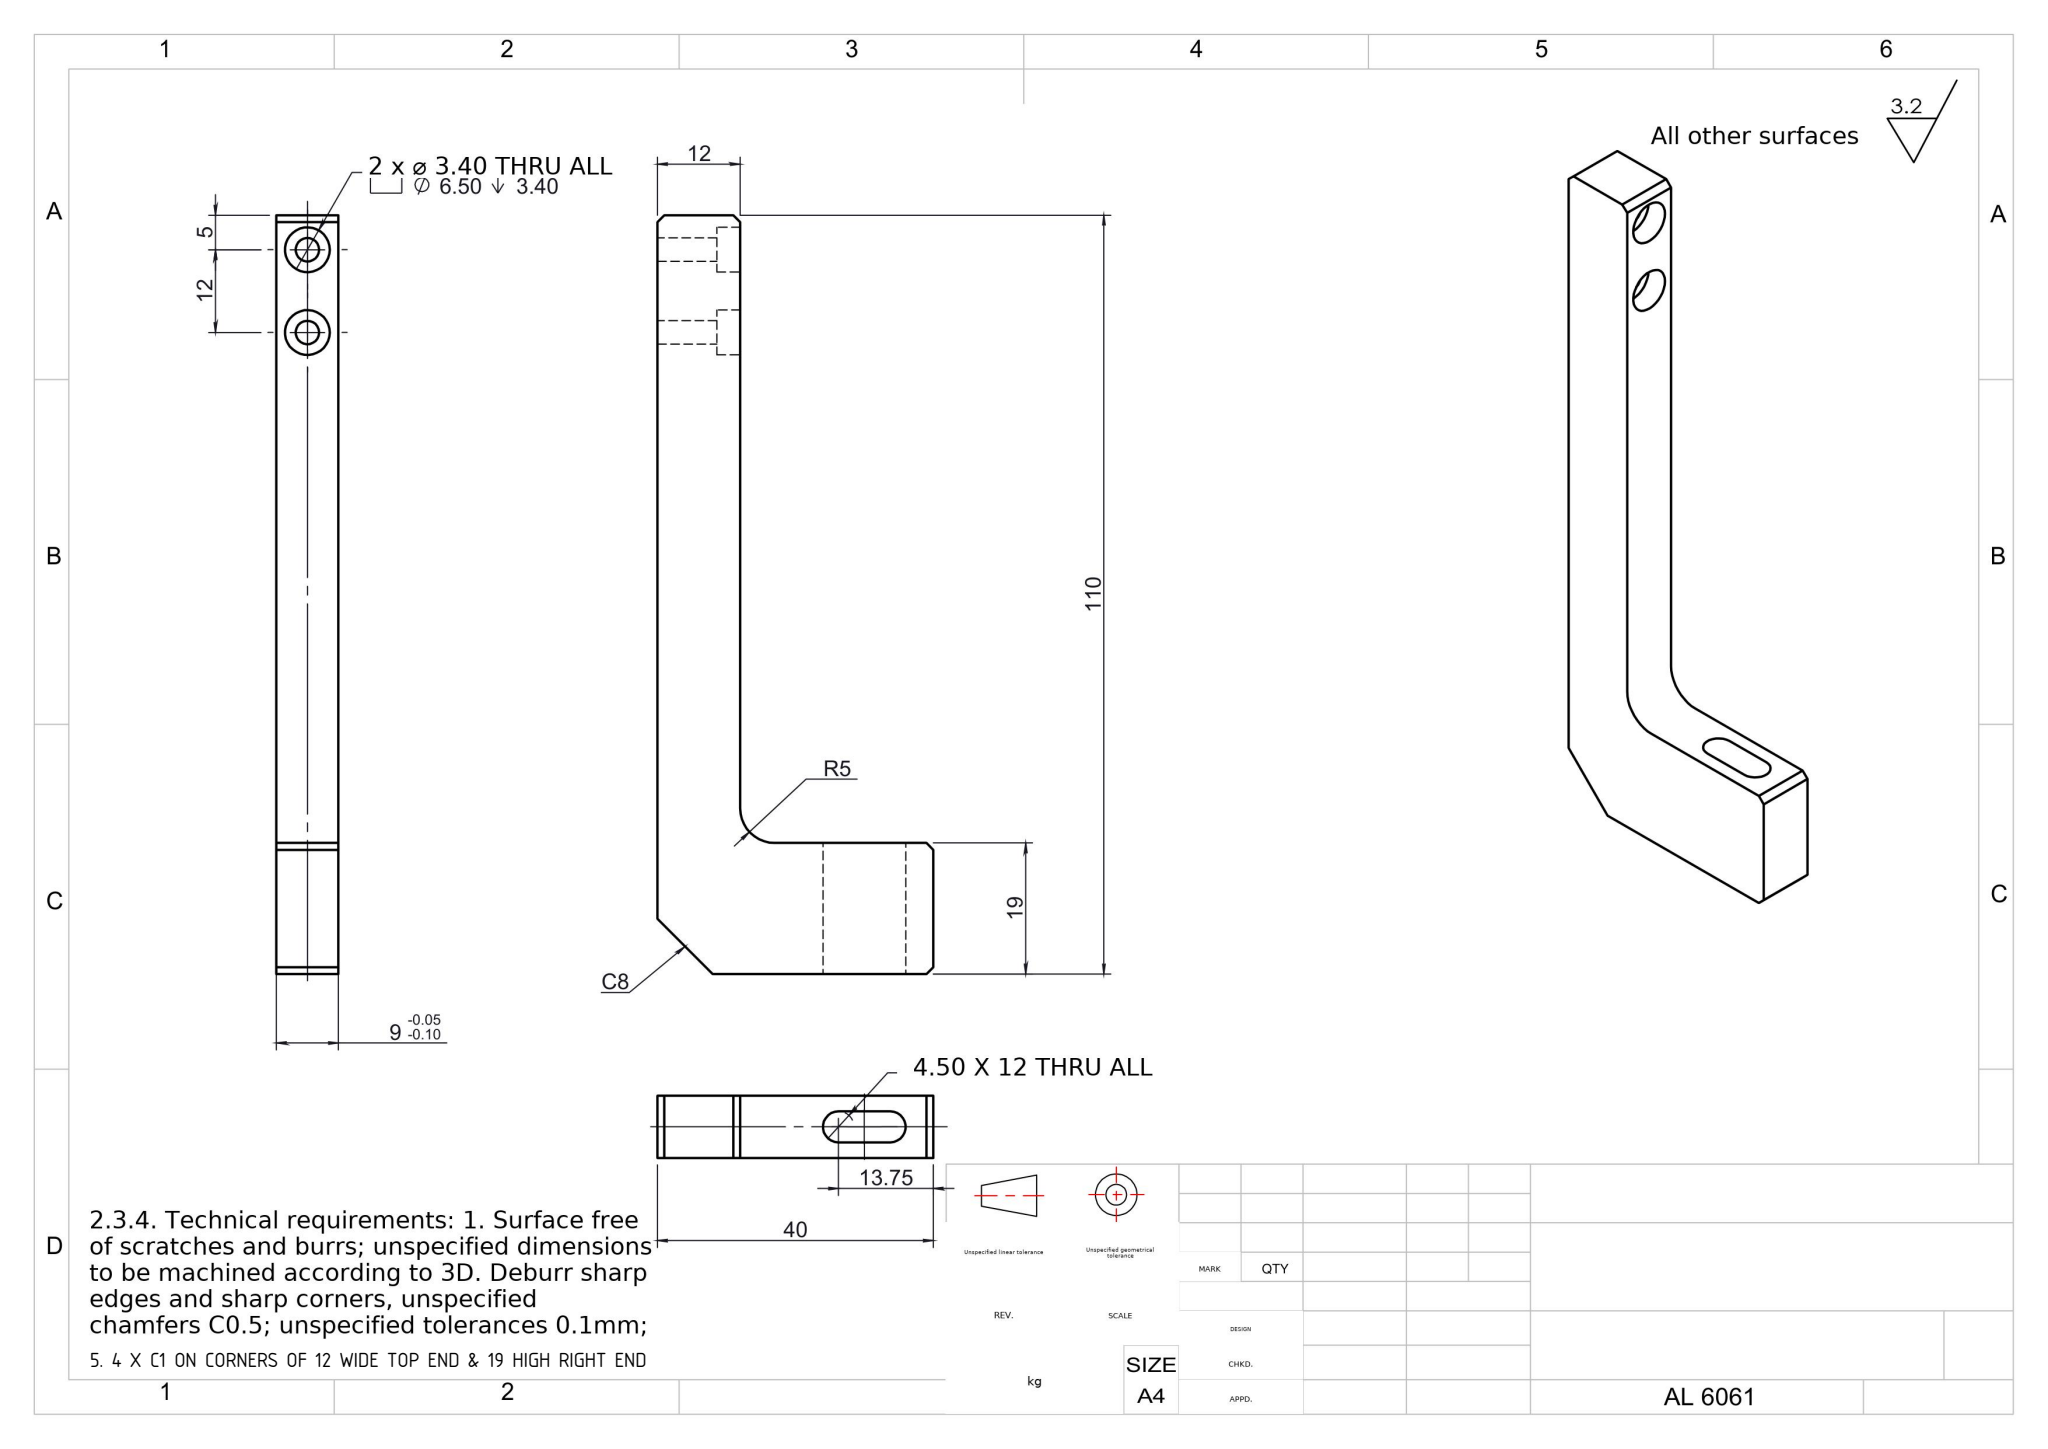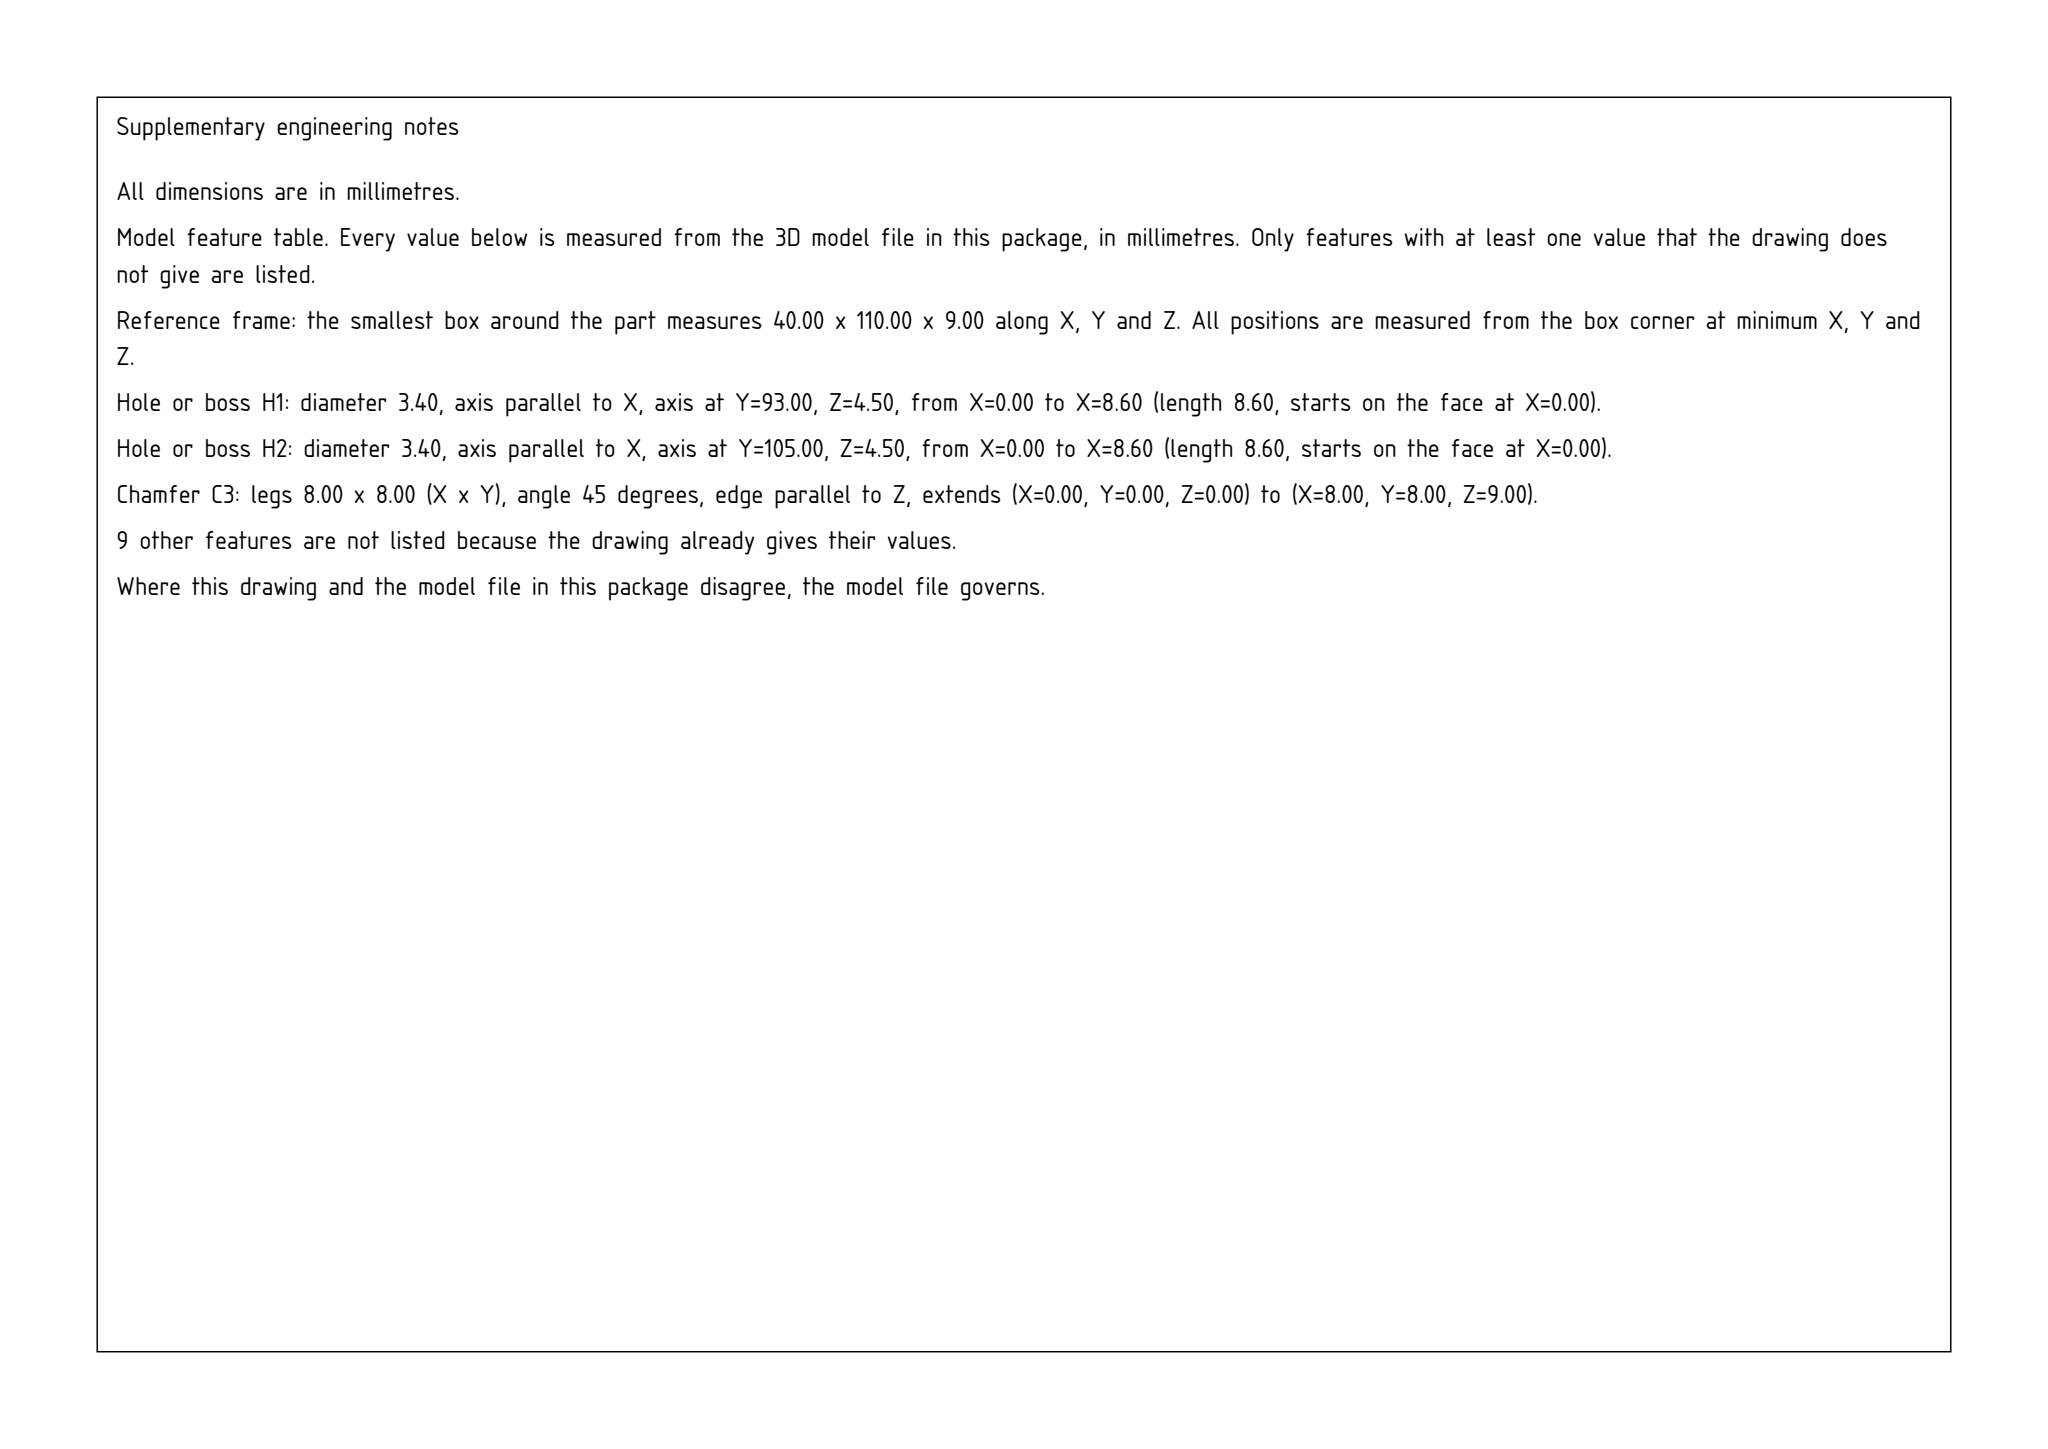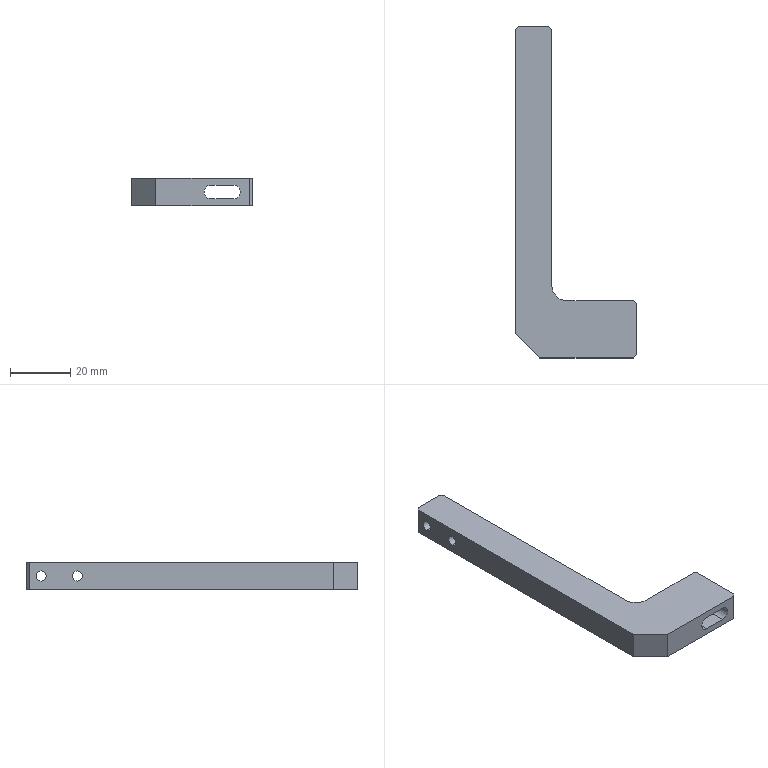Part | SolidWorks | mm | material AL 6061 | 1 solid | 28 faces | box 40 x 110 x 9 mm | volume 15085 mm3 | plane 17 | cylinder 11 | commonest cylinder face diameters 6.5 x4 3.4 x4 4.5 x2 10 x1
Drawing notes:
4 X C1 ON CORNERS OF 12 WIDE TOP END & 19 HIGH RIGHT END | from the solid: Four 45 deg inclined planes size 1x1x9 at [0,109,0], [11,109,0], [39,0,0], [39,18,0]; part bbox 40 x 110 x 9
STEP:
#1=CARTESIAN_POINT('',(-11.4,50.,3.25));
#2=VERTEX_POINT('',#1);
#3=CARTESIAN_POINT('',(-11.4,50.,-3.25));
#4=VERTEX_POINT('',#3);
#5=CARTESIAN_POINT('',(-11.4,50.,0.));
#6=DIRECTION('',(1.,0.,0.));
#7=DIRECTION('',(0.,0.,-1.));
#8=AXIS2_PLACEMENT_3D('',#5,#6,#7);
#9=CIRCLE('',#8,3.25);
#10=EDGE_CURVE('',#2,#4,#9,.T.);
#11=ORIENTED_EDGE('',*,*,#10,.F.);
#12=CARTESIAN_POINT('',(-8.,50.,3.25));
#13=VERTEX_POINT('',#12);
#14=CARTESIAN_POINT('',(-8.,50.,3.25));
#15=DIRECTION('',(1.,0.,0.));
#16=VECTOR('',#15,1000.);
#17=LINE('',#14,#16);
#18=EDGE_CURVE('',#2,#13,#17,.T.);
#19=ORIENTED_EDGE('',*,*,#18,.T.);
#20=CARTESIAN_POINT('',(-8.,50.,-3.25));
#21=VERTEX_POINT('',#20);
#22=CARTESIAN_POINT('',(-8.,50.,0.));
#23=DIRECTION('',(1.,0.,0.));
#24=DIRECTION('',(0.,0.,-1.));
#25=AXIS2_PLACEMENT_3D('',#22,#23,#24);
#26=CIRCLE('',#25,3.25);
#27=EDGE_CURVE('',#13,#21,#26,.T.);
#28=ORIENTED_EDGE('',*,*,#27,.T.);
#29=CARTESIAN_POINT('',(-8.,50.,-3.25));
#30=DIRECTION('',(1.,0.,0.));
#31=VECTOR('',#30,1000.);
#32=LINE('',#29,#31);
#33=EDGE_CURVE('',#4,#21,#32,.T.);
#34=ORIENTED_EDGE('',*,*,#33,.F.);
#35=EDGE_LOOP('',(#11,#19,#28,#34));
#36=FACE_OUTER_BOUND('',#35,.T.);
#37=CARTESIAN_POINT('',(-8.,50.,0.));
#38=DIRECTION('',(1.,0.,0.));
#39=DIRECTION('',(0.,0.,-1.));
#40=AXIS2_PLACEMENT_3D('',#37,#38,#39);
#41=CYLINDRICAL_SURFACE('',#40,3.25);
#42=ADVANCED_FACE('',(#36),#41,.F.);
#43=CARTESIAN_POINT('',(-20.,50.,1.7));
#44=VERTEX_POINT('',#43);
#45=CARTESIAN_POINT('',(-20.,50.,-1.7));
#46=VERTEX_POINT('',#45);
#47=CARTESIAN_POINT('',(-20.,50.,0.));
#48=DIRECTION('',(1.,0.,0.));
#49=DIRECTION('',(0.,0.,-1.));
#50=AXIS2_PLACEMENT_3D('',#47,#48,#49);
#51=CIRCLE('',#50,1.7);
#52=EDGE_CURVE('',#44,#46,#51,.T.);
#53=ORIENTED_EDGE('',*,*,#52,.F.);
#54=CARTESIAN_POINT('',(-11.4,50.,1.7));
#55=VERTEX_POINT('',#54);
#56=CARTESIAN_POINT('',(-8.,50.,1.7));
#57=DIRECTION('',(1.,0.,0.));
#58=VECTOR('',#57,1000.);
#59=LINE('',#56,#58);
#60=EDGE_CURVE('',#44,#55,#59,.T.);
#61=ORIENTED_EDGE('',*,*,#60,.T.);
#62=CARTESIAN_POINT('',(-11.4,50.,-1.7));
#63=VERTEX_POINT('',#62);
#64=CARTESIAN_POINT('',(-11.4,50.,0.));
#65=DIRECTION('',(1.,0.,0.));
#66=DIRECTION('',(0.,0.,-1.));
#67=AXIS2_PLACEMENT_3D('',#64,#65,#66);
#68=CIRCLE('',#67,1.7);
#69=EDGE_CURVE('',#55,#63,#68,.T.);
#70=ORIENTED_EDGE('',*,*,#69,.T.);
#71=CARTESIAN_POINT('',(-8.,50.,-1.7));
#72=DIRECTION('',(1.,0.,0.));
#73=VECTOR('',#72,1000.);
#74=LINE('',#71,#73);
#75=EDGE_CURVE('',#46,#63,#74,.T.);
#76=ORIENTED_EDGE('',*,*,#75,.F.);
#77=EDGE_LOOP('',(#53,#61,#70,#76));
#78=FACE_OUTER_BOUND('',#77,.T.);
#79=CARTESIAN_POINT('',(-8.,50.,0.));
#80=DIRECTION('',(1.,0.,0.));
#81=DIRECTION('',(0.,0.,-1.));
#82=AXIS2_PLACEMENT_3D('',#79,#80,#81);
#83=CYLINDRICAL_SURFACE('',#82,1.7);
#84=ADVANCED_FACE('',(#78),#83,.F.);
#85=CARTESIAN_POINT('',(-11.4,38.,3.25));
#86=VERTEX_POINT('',#85);
#87=CARTESIAN_POINT('',(-11.4,38.,-3.25));
#88=VERTEX_POINT('',#87);
#89=CARTESIAN_POINT('',(-11.4,38.,0.));
#90=DIRECTION('',(1.,0.,0.));
#91=DIRECTION('',(0.,0.,-1.));
#92=AXIS2_PLACEMENT_3D('',#89,#90,#91);
#93=CIRCLE('',#92,3.25);
#94=EDGE_CURVE('',#86,#88,#93,.T.);
#95=ORIENTED_EDGE('',*,*,#94,.F.);
#96=CARTESIAN_POINT('',(-8.,38.,3.25));
#97=VERTEX_POINT('',#96);
#98=CARTESIAN_POINT('',(-8.,38.,3.25));
#99=DIRECTION('',(1.,0.,0.));
#100=VECTOR('',#99,1000.);
#101=LINE('',#98,#100);
#102=EDGE_CURVE('',#86,#97,#101,.T.);
#103=ORIENTED_EDGE('',*,*,#102,.T.);
#104=CARTESIAN_POINT('',(-8.,38.,-3.25));
#105=VERTEX_POINT('',#104);
#106=CARTESIAN_POINT('',(-8.,38.,0.));
#107=DIRECTION('',(1.,0.,0.));
#108=DIRECTION('',(0.,0.,-1.));
#109=AXIS2_PLACEMENT_3D('',#106,#107,#108);
#110=CIRCLE('',#109,3.25);
#111=EDGE_CURVE('',#97,#105,#110,.T.);
#112=ORIENTED_EDGE('',*,*,#111,.T.);
#113=CARTESIAN_POINT('',(-8.,38.,-3.25));
#114=DIRECTION('',(1.,0.,0.));
#115=VECTOR('',#114,1000.);
#116=LINE('',#113,#115);
#117=EDGE_CURVE('',#88,#105,#116,.T.);
#118=ORIENTED_EDGE('',*,*,#117,.F.);
#119=EDGE_LOOP('',(#95,#103,#112,#118));
#120=FACE_OUTER_BOUND('',#119,.T.);
#121=CARTESIAN_POINT('',(-8.,38.,0.));
#122=DIRECTION('',(1.,0.,0.));
#123=DIRECTION('',(0.,0.,-1.));
#124=AXIS2_PLACEMENT_3D('',#121,#122,#123);
#125=CYLINDRICAL_SURFACE('',#124,3.25);
#126=ADVANCED_FACE('',(#120),#125,.F.);
#127=CARTESIAN_POINT('',(-20.,38.,1.7));
#128=VERTEX_POINT('',#127);
#129=CARTESIAN_POINT('',(-20.,38.,-1.7));
#130=VERTEX_POINT('',#129);
#131=CARTESIAN_POINT('',(-20.,38.,0.));
#132=DIRECTION('',(1.,0.,0.));
#133=DIRECTION('',(0.,0.,-1.));
#134=AXIS2_PLACEMENT_3D('',#131,#132,#133);
#135=CIRCLE('',#134,1.7);
#136=EDGE_CURVE('',#128,#130,#135,.T.);
#137=ORIENTED_EDGE('',*,*,#136,.F.);
#138=CARTESIAN_POINT('',(-11.4,38.,1.7));
#139=VERTEX_POINT('',#138);
#140=CARTESIAN_POINT('',(-8.,38.,1.7));
#141=DIRECTION('',(1.,0.,0.));
#142=VECTOR('',#141,1000.);
#143=LINE('',#140,#142);
#144=EDGE_CURVE('',#128,#139,#143,.T.);
#145=ORIENTED_EDGE('',*,*,#144,.T.);
#146=CARTESIAN_POINT('',(-11.4,38.,-1.7));
#147=VERTEX_POINT('',#146);
#148=CARTESIAN_POINT('',(-11.4,38.,0.));
#149=DIRECTION('',(1.,0.,0.));
#150=DIRECTION('',(0.,0.,-1.));
#151=AXIS2_PLACEMENT_3D('',#148,#149,#150);
#152=CIRCLE('',#151,1.7);
#153=EDGE_CURVE('',#139,#147,#152,.T.);
#154=ORIENTED_EDGE('',*,*,#153,.T.);
#155=CARTESIAN_POINT('',(-8.,38.,-1.7));
#156=DIRECTION('',(1.,0.,0.));
#157=VECTOR('',#156,1000.);
#158=LINE('',#155,#157);
#159=EDGE_CURVE('',#130,#147,#158,.T.);
#160=ORIENTED_EDGE('',*,*,#159,.F.);
#161=EDGE_LOOP('',(#137,#145,#154,#160));
#162=FACE_OUTER_BOUND('',#161,.T.);
#163=CARTESIAN_POINT('',(-8.,38.,0.));
#164=DIRECTION('',(1.,0.,0.));
#165=DIRECTION('',(0.,0.,-1.));
#166=AXIS2_PLACEMENT_3D('',#163,#164,#165);
#167=CYLINDRICAL_SURFACE('',#166,1.7);
#168=ADVANCED_FACE('',(#162),#167,.F.);
#169=CARTESIAN_POINT('',(-20.,50.,0.));
#170=DIRECTION('',(1.,0.,0.));
#171=DIRECTION('',(0.,0.,-1.));
#172=AXIS2_PLACEMENT_3D('',#169,#170,#171);
#173=CIRCLE('',#172,1.7);
#174=EDGE_CURVE('',#46,#44,#173,.T.);
#175=ORIENTED_EDGE('',*,*,#174,.T.);
#176=ORIENTED_EDGE('',*,*,#52,.T.);
#177=EDGE_LOOP('',(#175,#176));
#178=FACE_BOUND('',#177,.T.);
#179=CARTESIAN_POINT('',(-20.,38.,0.));
#180=DIRECTION('',(1.,0.,0.));
#181=DIRECTION('',(0.,0.,-1.));
#182=AXIS2_PLACEMENT_3D('',#179,#180,#181);
#183=CIRCLE('',#182,1.7);
#184=EDGE_CURVE('',#130,#128,#183,.T.);
#185=ORIENTED_EDGE('',*,*,#184,.T.);
#186=ORIENTED_EDGE('',*,*,#136,.T.);
#187=EDGE_LOOP('',(#185,#186));
#188=FACE_BOUND('',#187,.T.);
#189=CARTESIAN_POINT('',(-20.,54.,4.5));
#190=VERTEX_POINT('',#189);
#191=CARTESIAN_POINT('',(-20.,-47.,4.5));
#192=VERTEX_POINT('',#191);
#193=CARTESIAN_POINT('',(-20.,-55.,4.5));
#194=DIRECTION('',(0.,-1.,0.));
#195=VECTOR('',#194,1000.);
#196=LINE('',#193,#195);
#197=EDGE_CURVE('',#190,#192,#196,.T.);
#198=ORIENTED_EDGE('',*,*,#197,.F.);
#199=CARTESIAN_POINT('',(-20.,54.,-4.5));
#200=VERTEX_POINT('',#199);
#201=CARTESIAN_POINT('',(-20.,54.,4.5));
#202=DIRECTION('',(0.,0.,-1.));
#203=VECTOR('',#202,1000.);
#204=LINE('',#201,#203);
#205=EDGE_CURVE('',#190,#200,#204,.T.);
#206=ORIENTED_EDGE('',*,*,#205,.T.);
#207=CARTESIAN_POINT('',(-20.,-47.,-4.5));
#208=VERTEX_POINT('',#207);
#209=CARTESIAN_POINT('',(-20.,-55.,-4.5));
#210=DIRECTION('',(0.,-1.,0.));
#211=VECTOR('',#210,1000.);
#212=LINE('',#209,#211);
#213=EDGE_CURVE('',#200,#208,#212,.T.);
#214=ORIENTED_EDGE('',*,*,#213,.T.);
#215=CARTESIAN_POINT('',(-20.,-47.,4.5));
#216=DIRECTION('',(0.,0.,1.));
#217=VECTOR('',#216,1000.);
#218=LINE('',#215,#217);
#219=EDGE_CURVE('',#208,#192,#218,.T.);
#220=ORIENTED_EDGE('',*,*,#219,.T.);
#221=EDGE_LOOP('',(#198,#206,#214,#220));
#222=FACE_OUTER_BOUND('',#221,.T.);
#223=CARTESIAN_POINT('',(-20.,-55.,4.5));
#224=DIRECTION('',(1.,0.,0.));
#225=DIRECTION('',(0.,0.,-1.));
#226=AXIS2_PLACEMENT_3D('',#223,#224,#225);
#227=PLANE('',#226);
#228=ADVANCED_FACE('',(#178,#188,#222),#227,.F.);
#229=CARTESIAN_POINT('',(6.25,-55.,-2.25));
#230=VERTEX_POINT('',#229);
#231=CARTESIAN_POINT('',(6.25,-55.,2.25));
#232=VERTEX_POINT('',#231);
#233=CARTESIAN_POINT('',(6.25,-55.,-0.));
#234=DIRECTION('',(0.,1.,0.));
#235=DIRECTION('',(0.,0.,1.));
#236=AXIS2_PLACEMENT_3D('',#233,#234,#235);
#237=CIRCLE('',#236,2.25);
#238=EDGE_CURVE('',#230,#232,#237,.T.);
#239=ORIENTED_EDGE('',*,*,#238,.T.);
#240=CARTESIAN_POINT('',(13.75,-55.,2.25));
#241=VERTEX_POINT('',#240);
#242=CARTESIAN_POINT('',(6.25,-55.,2.25));
#243=DIRECTION('',(1.,0.,-0.));
#244=VECTOR('',#243,1000.);
#245=LINE('',#242,#244);
#246=EDGE_CURVE('',#232,#241,#245,.T.);
#247=ORIENTED_EDGE('',*,*,#246,.T.);
#248=CARTESIAN_POINT('',(13.75,-55.,-2.25));
#249=VERTEX_POINT('',#248);
#250=CARTESIAN_POINT('',(13.75,-55.,-0.));
#251=DIRECTION('',(0.,1.,0.));
#252=DIRECTION('',(0.,0.,1.));
#253=AXIS2_PLACEMENT_3D('',#250,#251,#252);
#254=CIRCLE('',#253,2.25);
#255=EDGE_CURVE('',#241,#249,#254,.T.);
#256=ORIENTED_EDGE('',*,*,#255,.T.);
#257=CARTESIAN_POINT('',(6.25,-55.,-2.25));
#258=DIRECTION('',(1.,0.,-0.));
#259=VECTOR('',#258,1000.);
#260=LINE('',#257,#259);
#261=EDGE_CURVE('',#230,#249,#260,.T.);
#262=ORIENTED_EDGE('',*,*,#261,.F.);
#263=EDGE_LOOP('',(#239,#247,#256,#262));
#264=FACE_BOUND('',#263,.T.);
#265=CARTESIAN_POINT('',(-12.,-55.,-4.5));
#266=VERTEX_POINT('',#265);
#267=CARTESIAN_POINT('',(19.,-55.,-4.5));
#268=VERTEX_POINT('',#267);
#269=CARTESIAN_POINT('',(20.,-55.,-4.5));
#270=DIRECTION('',(1.,0.,0.));
#271=VECTOR('',#270,1000.);
#272=LINE('',#269,#271);
#273=EDGE_CURVE('',#266,#268,#272,.T.);
#274=ORIENTED_EDGE('',*,*,#273,.T.);
#275=CARTESIAN_POINT('',(19.,-55.,4.5));
#276=VERTEX_POINT('',#275);
#277=CARTESIAN_POINT('',(19.,-55.,4.5));
#278=DIRECTION('',(0.,0.,1.));
#279=VECTOR('',#278,1000.);
#280=LINE('',#277,#279);
#281=EDGE_CURVE('',#268,#276,#280,.T.);
#282=ORIENTED_EDGE('',*,*,#281,.T.);
#283=CARTESIAN_POINT('',(-12.,-55.,4.5));
#284=VERTEX_POINT('',#283);
#285=CARTESIAN_POINT('',(20.,-55.,4.5));
#286=DIRECTION('',(1.,0.,0.));
#287=VECTOR('',#286,1000.);
#288=LINE('',#285,#287);
#289=EDGE_CURVE('',#284,#276,#288,.T.);
#290=ORIENTED_EDGE('',*,*,#289,.F.);
#291=CARTESIAN_POINT('',(-12.,-55.,4.5));
#292=DIRECTION('',(0.,0.,-1.));
#293=VECTOR('',#292,1000.);
#294=LINE('',#291,#293);
#295=EDGE_CURVE('',#284,#266,#294,.T.);
#296=ORIENTED_EDGE('',*,*,#295,.T.);
#297=EDGE_LOOP('',(#274,#282,#290,#296));
#298=FACE_OUTER_BOUND('',#297,.T.);
#299=CARTESIAN_POINT('',(20.,-55.,4.5));
#300=DIRECTION('',(0.,1.,0.));
#301=DIRECTION('',(0.,0.,1.));
#302=AXIS2_PLACEMENT_3D('',#299,#300,#301);
#303=PLANE('',#302);
#304=ADVANCED_FACE('',(#264,#298),#303,.F.);
#305=CARTESIAN_POINT('',(20.,-54.,4.5));
#306=VERTEX_POINT('',#305);
#307=CARTESIAN_POINT('',(20.,-37.,4.5));
#308=VERTEX_POINT('',#307);
#309=CARTESIAN_POINT('',(20.,-55.,4.5));
#310=DIRECTION('',(0.,1.,0.));
#311=VECTOR('',#310,1000.);
#312=LINE('',#309,#311);
#313=EDGE_CURVE('',#306,#308,#312,.T.);
#314=ORIENTED_EDGE('',*,*,#313,.F.);
#315=CARTESIAN_POINT('',(20.,-54.,-4.5));
#316=VERTEX_POINT('',#315);
#317=CARTESIAN_POINT('',(20.,-54.,4.5));
#318=DIRECTION('',(0.,0.,-1.));
#319=VECTOR('',#318,1000.);
#320=LINE('',#317,#319);
#321=EDGE_CURVE('',#306,#316,#320,.T.);
#322=ORIENTED_EDGE('',*,*,#321,.T.);
#323=CARTESIAN_POINT('',(20.,-37.,-4.5));
#324=VERTEX_POINT('',#323);
#325=CARTESIAN_POINT('',(20.,-55.,-4.5));
#326=DIRECTION('',(0.,1.,0.));
#327=VECTOR('',#326,1000.);
#328=LINE('',#325,#327);
#329=EDGE_CURVE('',#316,#324,#328,.T.);
#330=ORIENTED_EDGE('',*,*,#329,.T.);
#331=CARTESIAN_POINT('',(20.,-37.,4.5));
#332=DIRECTION('',(0.,0.,1.));
#333=VECTOR('',#332,1000.);
#334=LINE('',#331,#333);
#335=EDGE_CURVE('',#324,#308,#334,.T.);
#336=ORIENTED_EDGE('',*,*,#335,.T.);
#337=EDGE_LOOP('',(#314,#322,#330,#336));
#338=FACE_OUTER_BOUND('',#337,.T.);
#339=CARTESIAN_POINT('',(20.,-55.,4.5));
#340=DIRECTION('',(-1.,0.,0.));
#341=DIRECTION('',(0.,0.,1.));
#342=AXIS2_PLACEMENT_3D('',#339,#340,#341);
#343=PLANE('',#342);
#344=ADVANCED_FACE('',(#338),#343,.F.);
#345=CARTESIAN_POINT('',(-9.,55.,-4.5));
#346=VERTEX_POINT('',#345);
#347=CARTESIAN_POINT('',(-19.,55.,-4.5));
#348=VERTEX_POINT('',#347);
#349=CARTESIAN_POINT('',(20.,55.,-4.5));
#350=DIRECTION('',(-1.,0.,0.));
#351=VECTOR('',#350,1000.);
#352=LINE('',#349,#351);
#353=EDGE_CURVE('',#346,#348,#352,.T.);
#354=ORIENTED_EDGE('',*,*,#353,.T.);
#355=CARTESIAN_POINT('',(-19.,55.,4.5));
#356=VERTEX_POINT('',#355);
#357=CARTESIAN_POINT('',(-19.,55.,4.5));
#358=DIRECTION('',(0.,0.,1.));
#359=VECTOR('',#358,1000.);
#360=LINE('',#357,#359);
#361=EDGE_CURVE('',#348,#356,#360,.T.);
#362=ORIENTED_EDGE('',*,*,#361,.T.);
#363=CARTESIAN_POINT('',(-9.,55.,4.5));
#364=VERTEX_POINT('',#363);
#365=CARTESIAN_POINT('',(20.,55.,4.5));
#366=DIRECTION('',(-1.,0.,0.));
#367=VECTOR('',#366,1000.);
#368=LINE('',#365,#367);
#369=EDGE_CURVE('',#364,#356,#368,.T.);
#370=ORIENTED_EDGE('',*,*,#369,.F.);
#371=CARTESIAN_POINT('',(-9.,55.,4.5));
#372=DIRECTION('',(0.,0.,-1.));
#373=VECTOR('',#372,1000.);
#374=LINE('',#371,#373);
#375=EDGE_CURVE('',#364,#346,#374,.T.);
#376=ORIENTED_EDGE('',*,*,#375,.T.);
#377=EDGE_LOOP('',(#354,#362,#370,#376));
#378=FACE_OUTER_BOUND('',#377,.T.);
#379=CARTESIAN_POINT('',(20.,55.,4.5));
#380=DIRECTION('',(0.,-1.,0.));
#381=DIRECTION('',(0.,0.,-1.));
#382=AXIS2_PLACEMENT_3D('',#379,#380,#381);
#383=PLANE('',#382);
#384=ADVANCED_FACE('',(#378),#383,.F.);
#385=ORIENTED_EDGE('',*,*,#289,.T.);
#386=CARTESIAN_POINT('',(37.,-37.,4.5));
#387=DIRECTION('',(0.7071,0.7071,0.));
#388=VECTOR('',#387,1000.);
#389=LINE('',#386,#388);
#390=EDGE_CURVE('',#276,#306,#389,.T.);
#391=ORIENTED_EDGE('',*,*,#390,.T.);
#392=ORIENTED_EDGE('',*,*,#313,.T.);
#393=CARTESIAN_POINT('',(19.,-36.,4.5));
#394=VERTEX_POINT('',#393);
#395=CARTESIAN_POINT('',(-8.5,-8.5,4.5));
#396=DIRECTION('',(-0.7071,0.7071,0.));
#397=VECTOR('',#396,1000.);
#398=LINE('',#395,#397);
#399=EDGE_CURVE('',#308,#394,#398,.T.);
#400=ORIENTED_EDGE('',*,*,#399,.T.);
#401=CARTESIAN_POINT('',(-3.,-36.,4.5));
#402=VERTEX_POINT('',#401);
#403=CARTESIAN_POINT('',(20.,-36.,4.5));
#404=DIRECTION('',(1.,0.,0.));
#405=VECTOR('',#404,1000.);
#406=LINE('',#403,#405);
#407=EDGE_CURVE('',#402,#394,#406,.T.);
#408=ORIENTED_EDGE('',*,*,#407,.F.);
#409=CARTESIAN_POINT('',(-8.,-31.,4.5));
#410=VERTEX_POINT('',#409);
#411=CARTESIAN_POINT('',(-3.,-31.,4.5));
#412=DIRECTION('',(0.,0.,-1.));
#413=DIRECTION('',(1.,0.,0.));
#414=AXIS2_PLACEMENT_3D('',#411,#412,#413);
#415=CIRCLE('',#414,5.);
#416=EDGE_CURVE('',#402,#410,#415,.T.);
#417=ORIENTED_EDGE('',*,*,#416,.T.);
#418=CARTESIAN_POINT('',(-8.,54.,4.5));
#419=VERTEX_POINT('',#418);
#420=CARTESIAN_POINT('',(-8.,55.,4.5));
#421=DIRECTION('',(0.,-1.,0.));
#422=VECTOR('',#421,1000.);
#423=LINE('',#420,#422);
#424=EDGE_CURVE('',#419,#410,#423,.T.);
#425=ORIENTED_EDGE('',*,*,#424,.F.);
#426=CARTESIAN_POINT('',(23.,23.,4.5));
#427=DIRECTION('',(-0.7071,0.7071,0.));
#428=VECTOR('',#427,1000.);
#429=LINE('',#426,#428);
#430=EDGE_CURVE('',#419,#364,#429,.T.);
#431=ORIENTED_EDGE('',*,*,#430,.T.);
#432=ORIENTED_EDGE('',*,*,#369,.T.);
#433=CARTESIAN_POINT('',(-37.,37.,4.5));
#434=DIRECTION('',(-0.7071,-0.7071,0.));
#435=VECTOR('',#434,1000.);
#436=LINE('',#433,#435);
#437=EDGE_CURVE('',#356,#190,#436,.T.);
#438=ORIENTED_EDGE('',*,*,#437,.T.);
#439=ORIENTED_EDGE('',*,*,#197,.T.);
#440=CARTESIAN_POINT('',(-33.5,-33.5,4.5));
#441=DIRECTION('',(0.7071,-0.7071,0.));
#442=VECTOR('',#441,1000.);
#443=LINE('',#440,#442);
#444=EDGE_CURVE('',#192,#284,#443,.T.);
#445=ORIENTED_EDGE('',*,*,#444,.T.);
#446=EDGE_LOOP('',(#385,#391,#392,#400,#408,#417,#425,#431,#432,#438,#439,#445));
#447=FACE_OUTER_BOUND('',#446,.T.);
#448=CARTESIAN_POINT('',(0.,0.,4.5));
#449=DIRECTION('',(0.,0.,1.));
#450=DIRECTION('',(1.,0.,0.));
#451=AXIS2_PLACEMENT_3D('',#448,#449,#450);
#452=PLANE('',#451);
#453=ADVANCED_FACE('',(#447),#452,.T.);
#454=ORIENTED_EDGE('',*,*,#329,.F.);
#455=CARTESIAN_POINT('',(20.,-54.,-4.5));
#456=DIRECTION('',(-0.7071,-0.7071,0.));
#457=VECTOR('',#456,1000.);
#458=LINE('',#455,#457);
#459=EDGE_CURVE('',#316,#268,#458,.T.);
#460=ORIENTED_EDGE('',*,*,#459,.T.);
#461=ORIENTED_EDGE('',*,*,#273,.F.);
#462=CARTESIAN_POINT('',(-12.,-55.,-4.5));
#463=DIRECTION('',(-0.7071,0.7071,0.));
#464=VECTOR('',#463,1000.);
#465=LINE('',#462,#464);
#466=EDGE_CURVE('',#266,#208,#465,.T.);
#467=ORIENTED_EDGE('',*,*,#466,.T.);
#468=ORIENTED_EDGE('',*,*,#213,.F.);
#469=CARTESIAN_POINT('',(-20.,54.,-4.5));
#470=DIRECTION('',(0.7071,0.7071,0.));
#471=VECTOR('',#470,1000.);
#472=LINE('',#469,#471);
#473=EDGE_CURVE('',#200,#348,#472,.T.);
#474=ORIENTED_EDGE('',*,*,#473,.T.);
#475=ORIENTED_EDGE('',*,*,#353,.F.);
#476=CARTESIAN_POINT('',(-8.,54.,-4.5));
#477=VERTEX_POINT('',#476);
#478=CARTESIAN_POINT('',(-8.,54.,-4.5));
#479=DIRECTION('',(0.7071,-0.7071,0.));
#480=VECTOR('',#479,1000.);
#481=LINE('',#478,#480);
#482=EDGE_CURVE('',#346,#477,#481,.T.);
#483=ORIENTED_EDGE('',*,*,#482,.T.);
#484=CARTESIAN_POINT('',(-8.,-31.,-4.5));
#485=VERTEX_POINT('',#484);
#486=CARTESIAN_POINT('',(-8.,55.,-4.5));
#487=DIRECTION('',(0.,-1.,0.));
#488=VECTOR('',#487,1000.);
#489=LINE('',#486,#488);
#490=EDGE_CURVE('',#477,#485,#489,.T.);
#491=ORIENTED_EDGE('',*,*,#490,.T.);
#492=CARTESIAN_POINT('',(-3.,-36.,-4.5));
#493=VERTEX_POINT('',#492);
#494=CARTESIAN_POINT('',(-3.,-31.,-4.5));
#495=DIRECTION('',(0.,0.,1.));
#496=DIRECTION('',(1.,0.,0.));
#497=AXIS2_PLACEMENT_3D('',#494,#495,#496);
#498=CIRCLE('',#497,5.);
#499=EDGE_CURVE('',#485,#493,#498,.T.);
#500=ORIENTED_EDGE('',*,*,#499,.T.);
#501=CARTESIAN_POINT('',(19.,-36.,-4.5));
#502=VERTEX_POINT('',#501);
#503=CARTESIAN_POINT('',(20.,-36.,-4.5));
#504=DIRECTION('',(1.,0.,0.));
#505=VECTOR('',#504,1000.);
#506=LINE('',#503,#505);
#507=EDGE_CURVE('',#493,#502,#506,.T.);
#508=ORIENTED_EDGE('',*,*,#507,.T.);
#509=CARTESIAN_POINT('',(20.,-37.,-4.5));
#510=DIRECTION('',(0.7071,-0.7071,0.));
#511=VECTOR('',#510,1000.);
#512=LINE('',#509,#511);
#513=EDGE_CURVE('',#502,#324,#512,.T.);
#514=ORIENTED_EDGE('',*,*,#513,.T.);
#515=EDGE_LOOP('',(#454,#460,#461,#467,#468,#474,#475,#483,#491,#500,#508,#514));
#516=FACE_OUTER_BOUND('',#515,.T.);
#517=CARTESIAN_POINT('',(0.,0.,-4.5));
#518=DIRECTION('',(0.,0.,1.));
#519=DIRECTION('',(1.,0.,0.));
#520=AXIS2_PLACEMENT_3D('',#517,#518,#519);
#521=PLANE('',#520);
#522=ADVANCED_FACE('',(#516),#521,.F.);
#523=CARTESIAN_POINT('',(6.25,-36.,-2.25));
#524=VERTEX_POINT('',#523);
#525=CARTESIAN_POINT('',(6.25,-36.,2.25));
#526=VERTEX_POINT('',#525);
#527=CARTESIAN_POINT('',(6.25,-36.,-0.));
#528=DIRECTION('',(0.,1.,0.));
#529=DIRECTION('',(0.,0.,1.));
#530=AXIS2_PLACEMENT_3D('',#527,#528,#529);
#531=CIRCLE('',#530,2.25);
#532=EDGE_CURVE('',#524,#526,#531,.T.);
#533=ORIENTED_EDGE('',*,*,#532,.F.);
#534=CARTESIAN_POINT('',(13.75,-36.,-2.25));
#535=VERTEX_POINT('',#534);
#536=CARTESIAN_POINT('',(6.25,-36.,-2.25));
#537=DIRECTION('',(1.,0.,-0.));
#538=VECTOR('',#537,1000.);
#539=LINE('',#536,#538);
#540=EDGE_CURVE('',#524,#535,#539,.T.);
#541=ORIENTED_EDGE('',*,*,#540,.T.);
#542=CARTESIAN_POINT('',(13.75,-36.,2.25));
#543=VERTEX_POINT('',#542);
#544=CARTESIAN_POINT('',(13.75,-36.,-0.));
#545=DIRECTION('',(0.,1.,0.));
#546=DIRECTION('',(0.,0.,1.));
#547=AXIS2_PLACEMENT_3D('',#544,#545,#546);
#548=CIRCLE('',#547,2.25);
#549=EDGE_CURVE('',#543,#535,#548,.T.);
#550=ORIENTED_EDGE('',*,*,#549,.F.);
#551=CARTESIAN_POINT('',(6.25,-36.,2.25));
#552=DIRECTION('',(1.,0.,-0.));
#553=VECTOR('',#552,1000.);
#554=LINE('',#551,#553);
#555=EDGE_CURVE('',#526,#543,#554,.T.);
#556=ORIENTED_EDGE('',*,*,#555,.F.);
#557=EDGE_LOOP('',(#533,#541,#550,#556));
#558=FACE_BOUND('',#557,.T.);
#559=ORIENTED_EDGE('',*,*,#407,.T.);
#560=CARTESIAN_POINT('',(19.,-36.,-4.5));
#561=DIRECTION('',(0.,0.,-1.));
#562=VECTOR('',#561,1000.);
#563=LINE('',#560,#562);
#564=EDGE_CURVE('',#394,#502,#563,.T.);
#565=ORIENTED_EDGE('',*,*,#564,.T.);
#566=ORIENTED_EDGE('',*,*,#507,.F.);
#567=CARTESIAN_POINT('',(-3.,-36.,4.5));
#568=DIRECTION('',(0.,0.,1.));
#569=VECTOR('',#568,1000.);
#570=LINE('',#567,#569);
#571=EDGE_CURVE('',#493,#402,#570,.T.);
#572=ORIENTED_EDGE('',*,*,#571,.T.);
#573=EDGE_LOOP('',(#559,#565,#566,#572));
#574=FACE_OUTER_BOUND('',#573,.T.);
#575=CARTESIAN_POINT('',(20.,-36.,-4.5));
#576=DIRECTION('',(0.,-1.,0.));
#577=DIRECTION('',(0.,0.,-1.));
#578=AXIS2_PLACEMENT_3D('',#575,#576,#577);
#579=PLANE('',#578);
#580=ADVANCED_FACE('',(#558,#574),#579,.F.);
#581=CARTESIAN_POINT('',(-8.,50.,0.));
#582=DIRECTION('',(1.,0.,0.));
#583=DIRECTION('',(0.,0.,-1.));
#584=AXIS2_PLACEMENT_3D('',#581,#582,#583);
#585=CIRCLE('',#584,3.25);
#586=EDGE_CURVE('',#21,#13,#585,.T.);
#587=ORIENTED_EDGE('',*,*,#586,.F.);
#588=ORIENTED_EDGE('',*,*,#27,.F.);
#589=EDGE_LOOP('',(#587,#588));
#590=FACE_BOUND('',#589,.T.);
#591=CARTESIAN_POINT('',(-8.,38.,0.));
#592=DIRECTION('',(1.,0.,0.));
#593=DIRECTION('',(0.,0.,-1.));
#594=AXIS2_PLACEMENT_3D('',#591,#592,#593);
#595=CIRCLE('',#594,3.25);
#596=EDGE_CURVE('',#105,#97,#595,.T.);
#597=ORIENTED_EDGE('',*,*,#596,.F.);
#598=ORIENTED_EDGE('',*,*,#111,.F.);
#599=EDGE_LOOP('',(#597,#598));
#600=FACE_BOUND('',#599,.T.);
#601=ORIENTED_EDGE('',*,*,#490,.F.);
#602=CARTESIAN_POINT('',(-8.,54.,-4.5));
#603=DIRECTION('',(0.,0.,1.));
#604=VECTOR('',#603,1000.);
#605=LINE('',#602,#604);
#606=EDGE_CURVE('',#477,#419,#605,.T.);
#607=ORIENTED_EDGE('',*,*,#606,.T.);
#608=ORIENTED_EDGE('',*,*,#424,.T.);
#609=CARTESIAN_POINT('',(-8.,-31.,-4.5));
#610=DIRECTION('',(0.,0.,-1.));
#611=VECTOR('',#610,1000.);
#612=LINE('',#609,#611);
#613=EDGE_CURVE('',#410,#485,#612,.T.);
#614=ORIENTED_EDGE('',*,*,#613,.T.);
#615=EDGE_LOOP('',(#601,#607,#608,#614));
#616=FACE_OUTER_BOUND('',#615,.T.);
#617=CARTESIAN_POINT('',(-8.,55.,-4.5));
#618=DIRECTION('',(-1.,-0.,0.));
#619=DIRECTION('',(0.,-1.,0.));
#620=AXIS2_PLACEMENT_3D('',#617,#618,#619);
#621=PLANE('',#620);
#622=ADVANCED_FACE('',(#590,#600,#616),#621,.F.);
#623=ORIENTED_EDGE('',*,*,#444,.F.);
#624=ORIENTED_EDGE('',*,*,#219,.F.);
#625=ORIENTED_EDGE('',*,*,#466,.F.);
#626=ORIENTED_EDGE('',*,*,#295,.F.);
#627=EDGE_LOOP('',(#623,#624,#625,#626));
#628=FACE_OUTER_BOUND('',#627,.T.);
#629=CARTESIAN_POINT('',(-12.,-55.,4.5));
#630=DIRECTION('',(0.7071,0.7071,0.));
#631=DIRECTION('',(0.,0.,-1.));
#632=AXIS2_PLACEMENT_3D('',#629,#630,#631);
#633=PLANE('',#632);
#634=ADVANCED_FACE('',(#628),#633,.F.);
#635=ORIENTED_EDGE('',*,*,#499,.F.);
#636=ORIENTED_EDGE('',*,*,#613,.F.);
#637=ORIENTED_EDGE('',*,*,#416,.F.);
#638=ORIENTED_EDGE('',*,*,#571,.F.);
#639=EDGE_LOOP('',(#635,#636,#637,#638));
#640=FACE_OUTER_BOUND('',#639,.T.);
#641=CARTESIAN_POINT('',(-3.,-31.,-4.5));
#642=DIRECTION('',(0.,0.,-1.));
#643=DIRECTION('',(-1.,0.,0.));
#644=AXIS2_PLACEMENT_3D('',#641,#642,#643);
#645=CYLINDRICAL_SURFACE('',#644,5.);
#646=ADVANCED_FACE('',(#640),#645,.F.);
#647=ORIENTED_EDGE('',*,*,#390,.F.);
#648=ORIENTED_EDGE('',*,*,#281,.F.);
#649=ORIENTED_EDGE('',*,*,#459,.F.);
#650=ORIENTED_EDGE('',*,*,#321,.F.);
#651=EDGE_LOOP('',(#647,#648,#649,#650));
#652=FACE_OUTER_BOUND('',#651,.T.);
#653=CARTESIAN_POINT('',(20.,-54.,4.5));
#654=DIRECTION('',(-0.7071,0.7071,0.));
#655=DIRECTION('',(0.,0.,-1.));
#656=AXIS2_PLACEMENT_3D('',#653,#654,#655);
#657=PLANE('',#656);
#658=ADVANCED_FACE('',(#652),#657,.F.);
#659=ORIENTED_EDGE('',*,*,#437,.F.);
#660=ORIENTED_EDGE('',*,*,#361,.F.);
#661=ORIENTED_EDGE('',*,*,#473,.F.);
#662=ORIENTED_EDGE('',*,*,#205,.F.);
#663=EDGE_LOOP('',(#659,#660,#661,#662));
#664=FACE_OUTER_BOUND('',#663,.T.);
#665=CARTESIAN_POINT('',(-20.,54.,4.5));
#666=DIRECTION('',(0.7071,-0.7071,0.));
#667=DIRECTION('',(0.,0.,-1.));
#668=AXIS2_PLACEMENT_3D('',#665,#666,#667);
#669=PLANE('',#668);
#670=ADVANCED_FACE('',(#664),#669,.F.);
#671=ORIENTED_EDGE('',*,*,#482,.F.);
#672=ORIENTED_EDGE('',*,*,#375,.F.);
#673=ORIENTED_EDGE('',*,*,#430,.F.);
#674=ORIENTED_EDGE('',*,*,#606,.F.);
#675=EDGE_LOOP('',(#671,#672,#673,#674));
#676=FACE_OUTER_BOUND('',#675,.T.);
#677=CARTESIAN_POINT('',(-8.,54.,-4.5));
#678=DIRECTION('',(-0.7071,-0.7071,0.));
#679=DIRECTION('',(0.,0.,1.));
#680=AXIS2_PLACEMENT_3D('',#677,#678,#679);
#681=PLANE('',#680);
#682=ADVANCED_FACE('',(#676),#681,.F.);
#683=ORIENTED_EDGE('',*,*,#513,.F.);
#684=ORIENTED_EDGE('',*,*,#564,.F.);
#685=ORIENTED_EDGE('',*,*,#399,.F.);
#686=ORIENTED_EDGE('',*,*,#335,.F.);
#687=EDGE_LOOP('',(#683,#684,#685,#686));
#688=FACE_OUTER_BOUND('',#687,.T.);
#689=CARTESIAN_POINT('',(20.,-37.,4.5));
#690=DIRECTION('',(-0.7071,-0.7071,0.));
#691=DIRECTION('',(0.,0.,1.));
#692=AXIS2_PLACEMENT_3D('',#689,#690,#691);
#693=PLANE('',#692);
#694=ADVANCED_FACE('',(#688),#693,.F.);
#695=ORIENTED_EDGE('',*,*,#144,.F.);
#696=ORIENTED_EDGE('',*,*,#184,.F.);
#697=ORIENTED_EDGE('',*,*,#159,.T.);
#698=CARTESIAN_POINT('',(-11.4,38.,0.));
#699=DIRECTION('',(1.,0.,0.));
#700=DIRECTION('',(0.,0.,-1.));
#701=AXIS2_PLACEMENT_3D('',#698,#699,#700);
#702=CIRCLE('',#701,1.7);
#703=EDGE_CURVE('',#147,#139,#702,.T.);
#704=ORIENTED_EDGE('',*,*,#703,.T.);
#705=EDGE_LOOP('',(#695,#696,#697,#704));
#706=FACE_OUTER_BOUND('',#705,.T.);
#707=CARTESIAN_POINT('',(-8.,38.,0.));
#708=DIRECTION('',(1.,0.,0.));
#709=DIRECTION('',(0.,0.,-1.));
#710=AXIS2_PLACEMENT_3D('',#707,#708,#709);
#711=CYLINDRICAL_SURFACE('',#710,1.7);
#712=ADVANCED_FACE('',(#706),#711,.F.);
#713=ORIENTED_EDGE('',*,*,#703,.F.);
#714=ORIENTED_EDGE('',*,*,#153,.F.);
#715=EDGE_LOOP('',(#713,#714));
#716=FACE_BOUND('',#715,.T.);
#717=CARTESIAN_POINT('',(-11.4,38.,0.));
#718=DIRECTION('',(1.,0.,0.));
#719=DIRECTION('',(0.,0.,-1.));
#720=AXIS2_PLACEMENT_3D('',#717,#718,#719);
#721=CIRCLE('',#720,3.25);
#722=EDGE_CURVE('',#88,#86,#721,.T.);
#723=ORIENTED_EDGE('',*,*,#722,.T.);
#724=ORIENTED_EDGE('',*,*,#94,.T.);
#725=EDGE_LOOP('',(#723,#724));
#726=FACE_OUTER_BOUND('',#725,.T.);
#727=CARTESIAN_POINT('',(-11.4,39.7,0.));
#728=DIRECTION('',(-1.,0.,0.));
#729=DIRECTION('',(0.,0.,1.));
#730=AXIS2_PLACEMENT_3D('',#727,#728,#729);
#731=PLANE('',#730);
#732=ADVANCED_FACE('',(#716,#726),#731,.F.);
#733=ORIENTED_EDGE('',*,*,#102,.F.);
#734=ORIENTED_EDGE('',*,*,#722,.F.);
#735=ORIENTED_EDGE('',*,*,#117,.T.);
#736=ORIENTED_EDGE('',*,*,#596,.T.);
#737=EDGE_LOOP('',(#733,#734,#735,#736));
#738=FACE_OUTER_BOUND('',#737,.T.);
#739=CARTESIAN_POINT('',(-8.,38.,0.));
#740=DIRECTION('',(1.,0.,0.));
#741=DIRECTION('',(0.,0.,-1.));
#742=AXIS2_PLACEMENT_3D('',#739,#740,#741);
#743=CYLINDRICAL_SURFACE('',#742,3.25);
#744=ADVANCED_FACE('',(#738),#743,.F.);
#745=ORIENTED_EDGE('',*,*,#60,.F.);
#746=ORIENTED_EDGE('',*,*,#174,.F.);
#747=ORIENTED_EDGE('',*,*,#75,.T.);
#748=CARTESIAN_POINT('',(-11.4,50.,0.));
#749=DIRECTION('',(1.,0.,0.));
#750=DIRECTION('',(0.,0.,-1.));
#751=AXIS2_PLACEMENT_3D('',#748,#749,#750);
#752=CIRCLE('',#751,1.7);
#753=EDGE_CURVE('',#63,#55,#752,.T.);
#754=ORIENTED_EDGE('',*,*,#753,.T.);
#755=EDGE_LOOP('',(#745,#746,#747,#754));
#756=FACE_OUTER_BOUND('',#755,.T.);
#757=CARTESIAN_POINT('',(-8.,50.,0.));
#758=DIRECTION('',(1.,0.,0.));
#759=DIRECTION('',(0.,0.,-1.));
#760=AXIS2_PLACEMENT_3D('',#757,#758,#759);
#761=CYLINDRICAL_SURFACE('',#760,1.7);
#762=ADVANCED_FACE('',(#756),#761,.F.);
#763=ORIENTED_EDGE('',*,*,#753,.F.);
#764=ORIENTED_EDGE('',*,*,#69,.F.);
#765=EDGE_LOOP('',(#763,#764));
#766=FACE_BOUND('',#765,.T.);
#767=CARTESIAN_POINT('',(-11.4,50.,0.));
#768=DIRECTION('',(1.,0.,0.));
#769=DIRECTION('',(0.,0.,-1.));
#770=AXIS2_PLACEMENT_3D('',#767,#768,#769);
#771=CIRCLE('',#770,3.25);
#772=EDGE_CURVE('',#4,#2,#771,.T.);
#773=ORIENTED_EDGE('',*,*,#772,.T.);
#774=ORIENTED_EDGE('',*,*,#10,.T.);
#775=EDGE_LOOP('',(#773,#774));
#776=FACE_OUTER_BOUND('',#775,.T.);
#777=CARTESIAN_POINT('',(-11.4,51.7,0.));
#778=DIRECTION('',(-1.,0.,0.));
#779=DIRECTION('',(0.,0.,1.));
#780=AXIS2_PLACEMENT_3D('',#777,#778,#779);
#781=PLANE('',#780);
#782=ADVANCED_FACE('',(#766,#776),#781,.F.);
#783=ORIENTED_EDGE('',*,*,#18,.F.);
#784=ORIENTED_EDGE('',*,*,#772,.F.);
#785=ORIENTED_EDGE('',*,*,#33,.T.);
#786=ORIENTED_EDGE('',*,*,#586,.T.);
#787=EDGE_LOOP('',(#783,#784,#785,#786));
#788=FACE_OUTER_BOUND('',#787,.T.);
#789=CARTESIAN_POINT('',(-8.,50.,0.));
#790=DIRECTION('',(1.,0.,0.));
#791=DIRECTION('',(0.,0.,-1.));
#792=AXIS2_PLACEMENT_3D('',#789,#790,#791);
#793=CYLINDRICAL_SURFACE('',#792,3.25);
#794=ADVANCED_FACE('',(#788),#793,.F.);
#795=ORIENTED_EDGE('',*,*,#255,.F.);
#796=CARTESIAN_POINT('',(13.75,-36.,2.25));
#797=DIRECTION('',(0.,-1.,0.));
#798=VECTOR('',#797,1000.);
#799=LINE('',#796,#798);
#800=EDGE_CURVE('',#543,#241,#799,.T.);
#801=ORIENTED_EDGE('',*,*,#800,.F.);
#802=ORIENTED_EDGE('',*,*,#549,.T.);
#803=CARTESIAN_POINT('',(13.75,-36.,-2.25));
#804=DIRECTION('',(0.,1.,0.));
#805=VECTOR('',#804,1000.);
#806=LINE('',#803,#805);
#807=EDGE_CURVE('',#249,#535,#806,.T.);
#808=ORIENTED_EDGE('',*,*,#807,.F.);
#809=EDGE_LOOP('',(#795,#801,#802,#808));
#810=FACE_OUTER_BOUND('',#809,.T.);
#811=CARTESIAN_POINT('',(13.75,-36.,-0.));
#812=DIRECTION('',(0.,1.,0.));
#813=DIRECTION('',(0.,0.,1.));
#814=AXIS2_PLACEMENT_3D('',#811,#812,#813);
#815=CYLINDRICAL_SURFACE('',#814,2.25);
#816=ADVANCED_FACE('',(#810),#815,.F.);
#817=ORIENTED_EDGE('',*,*,#532,.T.);
#818=CARTESIAN_POINT('',(6.25,-36.,2.25));
#819=DIRECTION('',(0.,1.,0.));
#820=VECTOR('',#819,1000.);
#821=LINE('',#818,#820);
#822=EDGE_CURVE('',#232,#526,#821,.T.);
#823=ORIENTED_EDGE('',*,*,#822,.F.);
#824=ORIENTED_EDGE('',*,*,#238,.F.);
#825=CARTESIAN_POINT('',(6.25,-36.,-2.25));
#826=DIRECTION('',(0.,-1.,0.));
#827=VECTOR('',#826,1000.);
#828=LINE('',#825,#827);
#829=EDGE_CURVE('',#524,#230,#828,.T.);
#830=ORIENTED_EDGE('',*,*,#829,.F.);
#831=EDGE_LOOP('',(#817,#823,#824,#830));
#832=FACE_OUTER_BOUND('',#831,.T.);
#833=CARTESIAN_POINT('',(6.25,-36.,-0.));
#834=DIRECTION('',(0.,1.,0.));
#835=DIRECTION('',(0.,0.,1.));
#836=AXIS2_PLACEMENT_3D('',#833,#834,#835);
#837=CYLINDRICAL_SURFACE('',#836,2.25);
#838=ADVANCED_FACE('',(#832),#837,.F.);
#839=ORIENTED_EDGE('',*,*,#807,.T.);
#840=ORIENTED_EDGE('',*,*,#540,.F.);
#841=ORIENTED_EDGE('',*,*,#829,.T.);
#842=ORIENTED_EDGE('',*,*,#261,.T.);
#843=EDGE_LOOP('',(#839,#840,#841,#842));
#844=FACE_OUTER_BOUND('',#843,.T.);
#845=CARTESIAN_POINT('',(6.25,-36.,-2.25));
#846=DIRECTION('',(-0.,0.,-1.));
#847=DIRECTION('',(-1.,0.,0.));
#848=AXIS2_PLACEMENT_3D('',#845,#846,#847);
#849=PLANE('',#848);
#850=ADVANCED_FACE('',(#844),#849,.F.);
#851=ORIENTED_EDGE('',*,*,#800,.T.);
#852=ORIENTED_EDGE('',*,*,#246,.F.);
#853=ORIENTED_EDGE('',*,*,#822,.T.);
#854=ORIENTED_EDGE('',*,*,#555,.T.);
#855=EDGE_LOOP('',(#851,#852,#853,#854));
#856=FACE_OUTER_BOUND('',#855,.T.);
#857=CARTESIAN_POINT('',(6.25,-36.,2.25));
#858=DIRECTION('',(0.,0.,1.));
#859=DIRECTION('',(1.,0.,-0.));
#860=AXIS2_PLACEMENT_3D('',#857,#858,#859);
#861=PLANE('',#860);
#862=ADVANCED_FACE('',(#856),#861,.F.);
#863=CLOSED_SHELL('',(#42,#84,#126,#168,#228,#304,#344,#384,#453,#522,#580,#622,#634,#646,#658,#670,#682,#694,#712,#732,#744,#762,#782,#794,#816,#838,#850,#862));
#864=MANIFOLD_SOLID_BREP('',#863);
#865=CARTESIAN_POINT('',(0.,0.,0.));
#866=DIRECTION('',(0.,0.,1.));
#867=DIRECTION('',(1.,0.,0.));
#868=AXIS2_PLACEMENT_3D('',#865,#866,#867);
#869=(LENGTH_UNIT()NAMED_UNIT(*)SI_UNIT(.MILLI.,.METRE.));
#870=UNCERTAINTY_MEASURE_WITH_UNIT(LENGTH_MEASURE(0.00001),#869,'','');
#871=(NAMED_UNIT(*)PLANE_ANGLE_UNIT()SI_UNIT($,.RADIAN.));
#872=(NAMED_UNIT(*)SI_UNIT($,.STERADIAN.)SOLID_ANGLE_UNIT());
#873=(GEOMETRIC_REPRESENTATION_CONTEXT(3)GLOBAL_UNCERTAINTY_ASSIGNED_CONTEXT((#870))GLOBAL_UNIT_ASSIGNED_CONTEXT((#869,#871,#872))REPRESENTATION_CONTEXT('',''));
#874=ADVANCED_BREP_SHAPE_REPRESENTATION('',(#864,#868),#873);